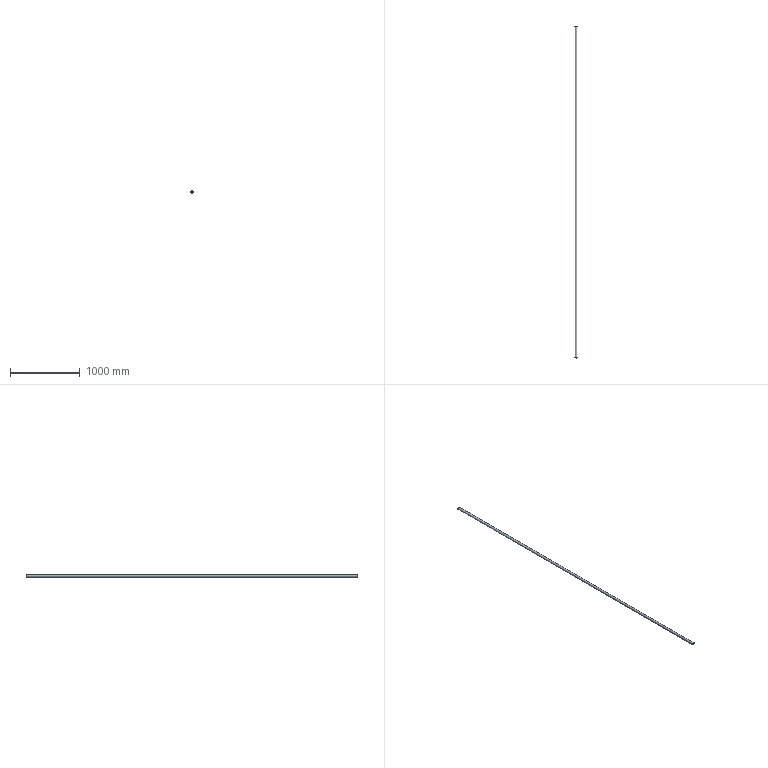Component | NX | 43_2_2 | 1 solid | 4 faces | volume 1592984 mm3 | cylinder 2 | plane 2 | commonest cylinder face diameters 34 x1 27 x1